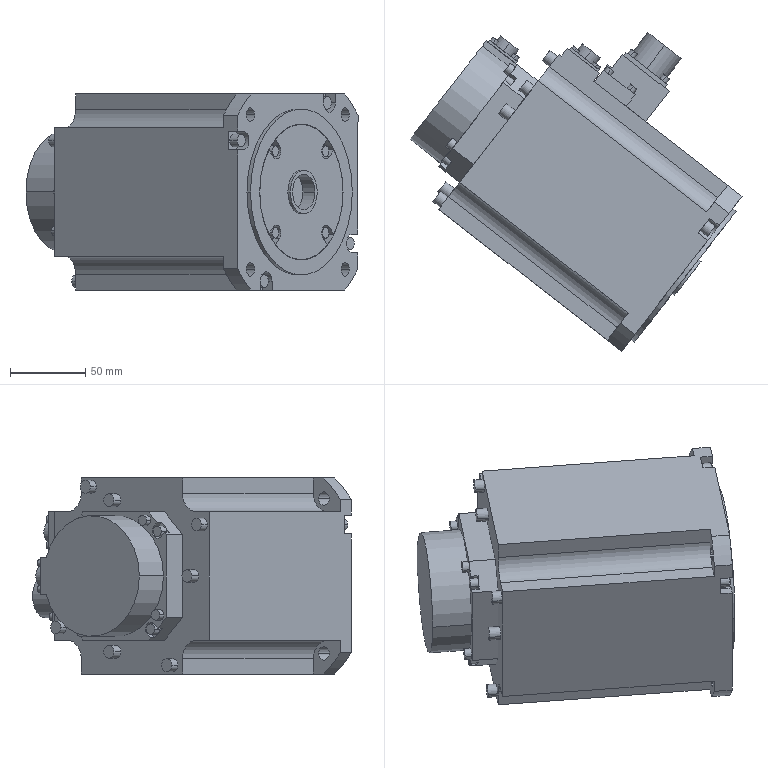Component | SolidWorks | 0803_102_Servo_Motor_850W-1_0803_Z_Servo_Motor_850W_1-1 | 1 solid | 270 faces | box 220 x 211.34 x 130 mm | volume 2662642 mm3 | plane 143 | cylinder 127 | commonest cylinder face diameters 7 x24 8.5 x22 5.5 x22 9 x14 4.95 x8 10 x6 24 x6 12.5 x5
build123d program:
from build123d import *

# Parameters (mm, degrees)
SKETCH1_W                = 130
SKETCH1_H                = 153.5
BOSS_EXTRUDE1_DEPTH      = 65
CUT_EXTRUDE1_DEPTH       = 141.5
BOSS_EXTRUDE2_DEPTH      = 17.5
BOSS_EXTRUDE3_DEPTH      = 26
SKETCH5_R                = 55
BOSS_EXTRUDE4_DEPTH      = 3
SKETCH6_R                = 45
CUT_EXTRUDE2_DEPTH       = 0.1
SKETCH7_R                = 14.5
BOSS_EXTRUDE5_DEPTH      = 2.1
SKETCH8_R                = 12
CUT_EXTRUDE3_DEPTH       = 10
CUT_EXTRUDE4_DEPTH       = 8
CUT_EXTRUDE5_DEPTH       = 5.6
SKETCH11_W               = 58
SKETCH11_H               = 26.6
BOSS_EXTRUDE6_DEPTH      = 9.8
SKETCH12_W               = 37.7
SKETCH12_H               = 42.9
BOSS_EXTRUDE7_DEPTH      = 25.5
SKETCH13_W               = 37.7
SKETCH13_H               = 3.7
CUT_EXTRUDE6_DEPTH       = 11
SKETCH14_W               = 34.9
SKETCH14_H               = 34.9
BOSS_EXTRUDE8_DEPTH      = 2.75
SKETCH15_R               = 14.2
BOSS_EXTRUDE9_DEPTH      = 19.25
SKETCH16_W               = 27
SKETCH16_H               = 27
BOSS_EXTRUDE10_DEPTH     = 6.5
SKETCH17_W               = 23.4
SKETCH17_H               = 23.4
BOSS_EXTRUDE11_DEPTH     = 1.7
SKETCH18_R               = 7.65
BOSS_EXTRUDE12_DEPTH     = 6.7
SKETCH19_W               = 23.4
SKETCH19_H               = 23.4
BOSS_EXTRUDE13_DEPTH     = 1.7
SKETCH20_R               = 7.65
BOSS_EXTRUDE14_DEPTH     = 6.7
CUT_EXTRUDE7_DEPTH       = 5
CUT_EXTRUDE8_DEPTH       = 227.067
SKETCH23_R               = 4.25
BOSS_EXTRUDE15_DEPTH     = 6.3
SKETCH24_R               = 4.25
BOSS_EXTRUDE16_DEPTH     = 7.5
SKETCH25_R               = 3.5
BOSS_EXTRUDE17_DEPTH     = 4.4
SKETCH26_R               = 3.5
BOSS_EXTRUDE18_DEPTH     = 5.5
SKETCH27_R               = 2.475
BOSS_EXTRUDE19_DEPTH     = 2.88
SKETCH28_R               = 2.795
SKETCH28_R_2             = 2.75
BOSS_EXTRUDE20_DEPTH     = 3.5
SKETCH29_R               = 2.75
BOSS_EXTRUDE21_DEPTH     = 3.75
SKETCH30_R               = 2.75
BOSS_EXTRUDE22_DEPTH     = 1.942
SKETCH31_R               = 4.25
BOSS_EXTRUDE23_DEPTH     = 6.3
SKETCH32_R               = 3.5
BOSS_EXTRUDE24_DEPTH     = 5
F_9_0_9_DIAMETER_HOLE1_D = 9


with BuildPart() as part:
    # Sketch1 → Boss-Extrude1 (new, symmetric)
    with BuildSketch(Plane.XY):
        with Locations((0, 76.75)):
            Rectangle(SKETCH1_W, SKETCH1_H)
    extrude(amount=BOSS_EXTRUDE1_DEPTH, both=True)

    # Sketch2 → Cut-Extrude1 (cut)
    with BuildSketch(Plane.XZ):
        with BuildLine():
            Line((-42.5, 65), (-42.5, 54.5))
            ThreePointArc((-42.5, 54.5), (-46.015, 46.015), (-54.5, 42.5))
            Line((-54.5, 42.5), (-65, 42.5))
            Line((-65, 42.5), (-65, 65))
            Line((-65, 65), (-42.5, 65))
        make_face()
        with BuildLine():
            Line((65, 65), (42.5, 65))
            Line((42.5, 65), (42.5, 54.5))
            ThreePointArc((42.5, 54.5), (46.015, 46.015), (54.5, 42.5))
            Line((54.5, 42.5), (65, 42.5))
            Line((65, 42.5), (65, 65))
        make_face()
        with BuildLine():
            Line((42.5, -65), (42.5, -54.5))
            ThreePointArc((42.5, -54.5), (46.015, -46.015), (54.5, -42.5))
            Line((54.5, -42.5), (65, -42.5))
            Line((65, -42.5), (65, -65))
            Line((65, -65), (42.5, -65))
        make_face()
        with BuildLine():
            Line((-65, -65), (-42.5, -65))
            Line((-42.5, -65), (-42.5, -54.5))
            ThreePointArc((-42.5, -54.5), (-46.015, -46.015), (-54.5, -42.5))
            Line((-54.5, -42.5), (-65, -42.5))
            Line((-65, -42.5), (-65, -65))
        make_face()
    extrude(amount=-CUT_EXTRUDE1_DEPTH, mode=Mode.SUBTRACT)

    # Sketch3 → Boss-Extrude2 (add)
    with BuildSketch(Plane.XZ):
        Polygon((-42.5, 27.5), (-27.5, 42.5), (27.5, 42.5), (42.5, 27.5), (42.5, -27.5), (27.5, -42.5), (-27.5, -42.5), (-42.5, -27.5), align=None)
    extrude(amount=BOSS_EXTRUDE2_DEPTH)

    # Sketch4 → Boss-Extrude3 (add)
    with BuildSketch(Plane.XZ.offset(17.5)):
        with BuildLine():
            Line((-12, -38.158), (-12, -42.5))
            Line((-12, -42.5), (12, -42.5))
            Line((12, -42.5), (12, -38.158))
            ThreePointArc((12, -38.158), (0, 40), (-12, -38.158))
        make_face()
    extrude(amount=BOSS_EXTRUDE3_DEPTH)

    # Sketch5 → Boss-Extrude4 (add)
    with BuildSketch(Plane(origin=(0, 153.5, 0), x_dir=(1, 0, 0), z_dir=(0, 1, 0))):
        with Locations(Location((0, 0, 0), (0, 0, 270))):
            Circle(SKETCH5_R)
    extrude(amount=BOSS_EXTRUDE4_DEPTH)

    # Sketch6 → Cut-Extrude2 (cut)
    with BuildSketch(Plane(origin=(0, 156.5, 0), x_dir=(1, 0, 0), z_dir=(0, 1, 0))):
        with Locations(Location((0, 0, 0), (0, 0, 270))):
            Circle(SKETCH6_R)
    extrude(amount=-CUT_EXTRUDE2_DEPTH, mode=Mode.SUBTRACT)

    # Sketch7 → Boss-Extrude5 (add)
    with BuildSketch(Plane(origin=(0, 156.4, 0), x_dir=(1, 0, 0), z_dir=(0, 1, 0))):
        with Locations(Location((0, 0, 0), (0, 0, 270))):
            Circle(SKETCH7_R)
    extrude(amount=BOSS_EXTRUDE5_DEPTH)

    # Sketch8 → Cut-Extrude3 (cut)
    with BuildSketch(Plane(origin=(0, 158.5, 0), x_dir=(1, 0, 0), z_dir=(0, 1, 0))):
        with Locations(Location((0, 0, 0), (0, 0, 270))):
            Circle(SKETCH8_R)
    extrude(amount=-CUT_EXTRUDE3_DEPTH, mode=Mode.SUBTRACT)

    # Sketch9 → Cut-Extrude4 (cut)
    with BuildSketch(Plane(origin=(0, 153.5, 0), x_dir=(1, 0, 0), z_dir=(0, 1, 0))):
        with BuildLine():
            Line((-40.35, -65), (-40.35, -59))
            ThreePointArc((-40.35, -59), (-34.1, -52.75), (-27.85, -59))
            Line((-27.85, -59), (-27.85, -65))
            Line((-27.85, -65), (-40.35, -65))
        make_face()
        with BuildLine():
            Line((-59, 27.85), (-65, 27.85))
            Line((-65, 27.85), (-65, 40.35))
            Line((-65, 40.35), (-59, 40.35))
            ThreePointArc((-59, 40.35), (-52.75, 34.1), (-59, 27.85))
        make_face()
        with BuildLine():
            Line((27.85, 59), (27.85, 65))
            Line((27.85, 65), (40.35, 65))
            Line((40.35, 65), (40.35, 59))
            ThreePointArc((40.35, 59), (34.1, 52.75), (27.85, 59))
        make_face()
        with BuildLine():
            Line((59, -27.85), (65, -27.85))
            Line((65, -27.85), (65, -40.35))
            Line((65, -40.35), (59, -40.35))
            ThreePointArc((59, -40.35), (52.75, -34.1), (59, -27.85))
        make_face()
    extrude(amount=-CUT_EXTRUDE4_DEPTH, mode=Mode.SUBTRACT)

    # Sketch10 → Cut-Extrude5 (cut)
    with BuildSketch(Plane(origin=(0, 156.4, 0), x_dir=(1, 0, 0), z_dir=(0, 1, 0))):
        with BuildLine():
            Line((-35.158, 28.087), (-30.582, 23.511))
            ThreePointArc((-30.582, 23.511), (-23.511, 23.511), (-23.511, 30.582))
            Line((-23.511, 30.582), (-28.087, 35.158))
            ThreePointArc((-28.087, 35.158), (-31.82, 31.82), (-35.158, 28.087))
        make_face()
        with BuildLine():
            Line((28.087, 35.158), (23.511, 30.582))
            ThreePointArc((23.511, 30.582), (23.511, 23.511), (30.582, 23.511))
            Line((30.582, 23.511), (35.158, 28.087))
            ThreePointArc((35.158, 28.087), (31.82, 31.82), (28.087, 35.158))
        make_face()
        with BuildLine():
            Line((35.158, -28.087), (30.582, -23.511))
            ThreePointArc((30.582, -23.511), (23.511, -23.511), (23.511, -30.582))
            Line((23.511, -30.582), (28.087, -35.158))
            ThreePointArc((28.087, -35.158), (31.82, -31.82), (35.158, -28.087))
        make_face()
        with BuildLine():
            Line((-28.087, -35.158), (-23.511, -30.582))
            ThreePointArc((-23.511, -30.582), (-23.511, -23.511), (-30.582, -23.511))
            Line((-30.582, -23.511), (-35.158, -28.087))
            ThreePointArc((-35.158, -28.087), (-31.82, -31.82), (-28.087, -35.158))
        make_face()
    extrude(amount=-CUT_EXTRUDE5_DEPTH, mode=Mode.SUBTRACT)

    # Sketch11 → Boss-Extrude6 (add)
    with BuildSketch(Plane(origin=(0, 0, -65), x_dir=(-1, 0, 0), z_dir=(0, 0, -1))):
        with Locations((-13.5, 43)):
            Rectangle(SKETCH11_W, SKETCH11_H)
    extrude(amount=BOSS_EXTRUDE6_DEPTH)

    # Sketch12 → Boss-Extrude7 (add)
    with BuildSketch(Plane(origin=(0, 0, -65), x_dir=(-1, 0, 0), z_dir=(0, 0, -1))):
        with Locations((-13.5, 51.15)):
            Rectangle(SKETCH12_W, SKETCH12_H)
    extrude(amount=BOSS_EXTRUDE7_DEPTH)

    # Sketch13 → Cut-Extrude6 (cut)
    with BuildSketch(Plane(origin=(0, 0, -90.5), x_dir=(-1, 0, 0), z_dir=(0, 0, -1))):
        with Locations((-13.5, 31.55)):
            Rectangle(SKETCH13_W, SKETCH13_H)
    extrude(amount=-CUT_EXTRUDE6_DEPTH, mode=Mode.SUBTRACT)

    # Sketch14 → Boss-Extrude8 (add)
    with BuildSketch(Plane(origin=(0, 0, -90.5), x_dir=(-1, 0, 0), z_dir=(0, 0, -1))):
        with Locations((-13.5, 51.7)):
            Rectangle(SKETCH14_W, SKETCH14_H)
    extrude(amount=BOSS_EXTRUDE8_DEPTH)

    # Sketch15 → Boss-Extrude9 (add)
    with BuildSketch(Plane(origin=(0, 0, -93.25), x_dir=(-1, 0, 0), z_dir=(0, 0, -1))):
        with Locations((-13.5, 51.7)):
            Circle(SKETCH15_R)
    extrude(amount=BOSS_EXTRUDE9_DEPTH)

    # Sketch16 → Boss-Extrude10 (add)
    with BuildSketch(Plane(origin=(0, 0, -65), x_dir=(-1, 0, 0), z_dir=(0, 0, -1))):
        with Locations((29, 15.5)):
            Rectangle(SKETCH16_W, SKETCH16_H)
    extrude(amount=BOSS_EXTRUDE10_DEPTH)

    # Sketch17 → Boss-Extrude11 (add)
    with BuildSketch(Plane(origin=(0, 0, -71.5), x_dir=(-1, 0, 0), z_dir=(0, 0, -1))):
        with Locations((29, 15.5)):
            Rectangle(SKETCH17_W, SKETCH17_H)
    extrude(amount=BOSS_EXTRUDE11_DEPTH)

    # Sketch18 → Boss-Extrude12 (add)
    with BuildSketch(Plane(origin=(0, 0, -73.2), x_dir=(-1, 0, 0), z_dir=(0, 0, -1))):
        with Locations((29, 15.5)):
            Circle(SKETCH18_R)
    extrude(amount=BOSS_EXTRUDE12_DEPTH)

    # Sketch19 → Boss-Extrude13 (add)
    with BuildSketch(Plane(origin=(0, 0, -42.5), x_dir=(-1, 0, 0), z_dir=(0, 0, -1))):
        with Locations((0, -30.5)):
            Rectangle(SKETCH19_W, SKETCH19_H)
    extrude(amount=BOSS_EXTRUDE13_DEPTH)

    # Sketch20 → Boss-Extrude14 (add)
    with BuildSketch(Plane(origin=(0, 0, -44.2), x_dir=(-1, 0, 0), z_dir=(0, 0, -1))):
        with Locations((0, -30.5)):
            Circle(SKETCH20_R)
    extrude(amount=BOSS_EXTRUDE14_DEPTH)

    # Sketch21 → Cut-Extrude7 (cut)
    with BuildSketch(Plane.XZ.offset(17.5)):
        with BuildLine():
            Line((-28.983, 41.017), (-26.386, 38.42))
            ThreePointArc((-26.386, 38.42), (-26.386, 32.056), (-32.75, 32.056))
            Line((-32.75, 32.056), (-35.347, 34.653))
            Line((-35.347, 34.653), (-28.983, 41.017))
        make_face()
        with BuildLine():
            Line((32.056, 32.75), (34.653, 35.347))
            Line((34.653, 35.347), (41.017, 28.983))
            Line((41.017, 28.983), (38.42, 26.386))
            ThreePointArc((38.42, 26.386), (32.056, 26.386), (32.056, 32.75))
        make_face()
        with BuildLine():
            Line((32.75, -32.056), (35.347, -34.653))
            Line((35.347, -34.653), (28.983, -41.017))
            Line((28.983, -41.017), (26.386, -38.42))
            ThreePointArc((26.386, -38.42), (26.386, -32.056), (32.75, -32.056))
        make_face()
        with BuildLine():
            Line((-32.056, -32.75), (-34.653, -35.347))
            Line((-34.653, -35.347), (-41.017, -28.983))
            Line((-41.017, -28.983), (-38.42, -26.386))
            ThreePointArc((-38.42, -26.386), (-32.056, -26.386), (-32.056, -32.75))
        make_face()
    extrude(amount=-CUT_EXTRUDE7_DEPTH, mode=Mode.SUBTRACT)

    # Sketch22 → Cut-Extrude8 (cut, through all)
    with BuildSketch(Plane.XZ.offset(-141.5)):
        with BuildLine():
            Line((65, 50.806), (65, 65))
            Line((65, 65), (50.806, 65))
            ThreePointArc((50.806, 65), (58.336, 58.336), (65, 50.806))
        make_face()
        with BuildLine():
            Line((-50.806, 65), (-65, 65))
            Line((-65, 65), (-65, 50.806))
            ThreePointArc((-65, 50.806), (-58.336, 58.336), (-50.806, 65))
        make_face()
        with BuildLine():
            Line((-65, -50.806), (-65, -65))
            Line((-65, -65), (-50.806, -65))
            ThreePointArc((-50.806, -65), (-58.336, -58.336), (-65, -50.806))
        make_face()
        with BuildLine():
            Line((50.806, -65), (65, -65))
            Line((65, -65), (65, -50.806))
            ThreePointArc((65, -50.806), (58.336, -58.336), (50.806, -65))
        make_face()
    extrude(amount=-CUT_EXTRUDE8_DEPTH, mode=Mode.SUBTRACT)

    # Sketch23 → Boss-Extrude15 (add)
    with BuildSketch(Plane.XZ):
        with Locations(Location((-34.1, 59.1, 0), (0, 0, 270))):
            Circle(SKETCH23_R)
        with Locations(Location((59.1, 34.1, 0), (0, 0, 270))):
            Circle(SKETCH23_R)
        with Locations(Location((34.1, -59.1, 0), (0, 0, 270))):
            Circle(SKETCH23_R)
        with Locations(Location((-59.1, -34.1, 0), (0, 0, 270))):
            Circle(SKETCH23_R)
    extrude(amount=BOSS_EXTRUDE15_DEPTH)

    # Sketch24 → Boss-Extrude16 (add)
    with BuildSketch(Plane.XZ):
        with Locations(Location((50.228, -13.459, 0), (0, 0, 270))):
            Circle(SKETCH24_R)
        with Locations(Location((0, 52, 0), (0, 0, 270))):
            Circle(SKETCH24_R)
        with Locations(Location((-50.228, -13.459, 0), (0, 0, 270))):
            Circle(SKETCH24_R)
    extrude(amount=BOSS_EXTRUDE16_DEPTH)

    # Sketch25 → Boss-Extrude17 (add)
    with BuildSketch(Plane.XZ.offset(17.5)):
        with Locations(Location((25.811, 36.862, 0), (0, 0, 90))):
            Circle(SKETCH25_R)
        with Locations(Location((36.862, -25.811, 0), (0, 0, 90))):
            Circle(SKETCH25_R)
        with Locations(Location((-25.811, -36.862, 0), (0, 0, 90))):
            Circle(SKETCH25_R)
        with Locations(Location((-36.862, 25.811, 0), (0, 0, 90))):
            Circle(SKETCH25_R)
    extrude(amount=BOSS_EXTRUDE17_DEPTH)

    # Sketch26 → Boss-Extrude18 (add)
    with BuildSketch(Plane.XZ.offset(12.5)):
        with Locations(Location((35.238, 29.568, 0), (0, 0, 90))):
            Circle(SKETCH26_R)
        with Locations(Location((29.568, -35.238, 0), (0, 0, 90))):
            Circle(SKETCH26_R)
        with Locations(Location((-35.238, -29.568, 0), (0, 0, 90))):
            Circle(SKETCH26_R)
        with Locations(Location((-29.568, 35.238, 0), (0, 0, 90))):
            Circle(SKETCH26_R)
    extrude(amount=BOSS_EXTRUDE18_DEPTH)

    # Sketch27 → Boss-Extrude19 (add)
    with BuildSketch(Plane(origin=(0, 0, -44.2), x_dir=(-1, 0, 0), z_dir=(0, 0, -1))):
        with Locations(Location((8.63, -21.87, 0), (0, 0, 180))):
            Circle(SKETCH27_R)
        with Locations(Location((8.63, -39.13, 0), (0, 0, 180))):
            Circle(SKETCH27_R)
        with Locations(Location((-8.63, -39.13, 0), (0, 0, 180))):
            Circle(SKETCH27_R)
        with Locations(Location((-8.63, -21.87, 0), (0, 0, 180))):
            Circle(SKETCH27_R)
    extrude(amount=BOSS_EXTRUDE19_DEPTH)

    # Sketch28 → Boss-Extrude20 (add)
    with BuildSketch(Plane(origin=(0, 0, -74.8), x_dir=(-1, 0, 0), z_dir=(0, 0, -1))):
        with Locations((12, 52)):
            Circle(SKETCH28_R)
        with Locations((12, 33)):
            Circle(SKETCH28_R_2)
        with Locations((-39, 33)):
            Circle(SKETCH28_R_2)
        with Locations((-39, 52)):
            Circle(SKETCH28_R_2)
    extrude(amount=BOSS_EXTRUDE20_DEPTH)

    # Sketch29 → Boss-Extrude21 (add)
    with BuildSketch(Plane(origin=(0, 0, -93.25), x_dir=(-1, 0, 0), z_dir=(0, 0, -1))):
        with Locations((-0.015, 65.185)):
            Circle(SKETCH29_R)
        with Locations((-0.015, 38.215)):
            Circle(SKETCH29_R)
        with Locations((-26.985, 38.215)):
            Circle(SKETCH29_R)
        with Locations((-26.985, 65.185)):
            Circle(SKETCH29_R)
    extrude(amount=BOSS_EXTRUDE21_DEPTH)

    # Sketch30 → Boss-Extrude22 (add)
    with BuildSketch(Plane(origin=(0, 0, -73.2), x_dir=(-1, 0, 0), z_dir=(0, 0, -1))):
        with Locations((37.63, 24.13)):
            Circle(SKETCH30_R)
        with Locations((37.63, 6.87)):
            Circle(SKETCH30_R)
        with Locations((20.37, 6.87)):
            Circle(SKETCH30_R)
        with Locations((20.37, 24.13)):
            Circle(SKETCH30_R)
    extrude(amount=BOSS_EXTRUDE22_DEPTH)

    # Sketch31 → Boss-Extrude23 (add)
    with BuildSketch(Plane(origin=(0, 145.5, 0), x_dir=(1, 0, 0), z_dir=(0, 1, 0))):
        with Locations(Location((34.1, 59, 0), (0, 0, 90))):
            Circle(SKETCH31_R)
        with Locations(Location((59, -34.1, 0), (0, 0, 90))):
            Circle(SKETCH31_R)
        with Locations(Location((-59, 34.1, 0), (0, 0, 90))):
            Circle(SKETCH31_R)
        with Locations(Location((-34.1, -59, 0), (0, 0, 90))):
            Circle(SKETCH31_R)
    extrude(amount=BOSS_EXTRUDE23_DEPTH)

    # Sketch32 → Boss-Extrude24 (add)
    with BuildSketch(Plane(origin=(0, 150.8, 0), x_dir=(1, 0, 0), z_dir=(0, 1, 0))):
        with Locations(Location((-27.047, 27.047, 0), (0, 0, 270))):
            Circle(SKETCH32_R)
        with Locations(Location((27.047, 27.047, 0), (0, 0, 270))):
            Circle(SKETCH32_R)
        with Locations(Location((27.047, -27.047, 0), (0, 0, 270))):
            Circle(SKETCH32_R)
        with Locations(Location((-27.047, -27.047, 0), (0, 0, 270))):
            Circle(SKETCH32_R)
    extrude(amount=BOSS_EXTRUDE24_DEPTH)

    # 9.0 _9_ Diameter Hole1 (through all)
    with Locations(Plane(origin=(0, 153.5, 0), x_dir=(-1, 0, 0), z_dir=(0, 1, 0))):
        with Locations((-51.265, 51.265), (51.265, 51.265), (51.265, -51.265), (-51.265, -51.265)):
            Hole(F_9_0_9_DIAMETER_HOLE1_D / 2)


solid = part.part

# Placed as in the assembly
solid = solid.moved(Location((-339.347, 1008.063, 276.411), (90, -37.821, -90)))